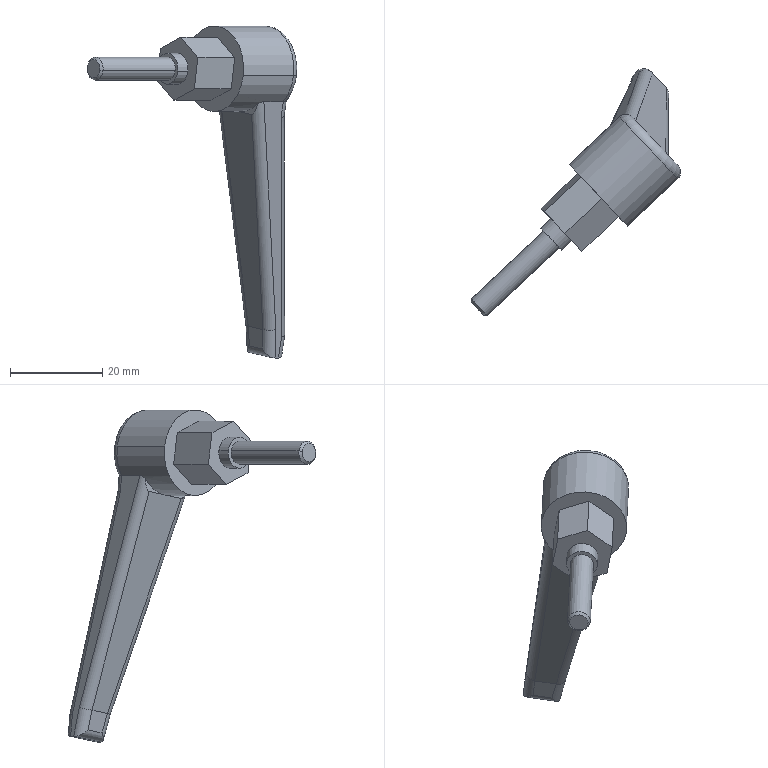Component | SolidWorks | M5AdjustableHandle-1 | 1 solid | 59 faces | volume 10442 mm3 | plane 34 | cylinder 20 | torus 3 | cone 2 | commonest cylinder face diameters 4 x12 18.6 x2 11 x2 6.7 x2 5 x2